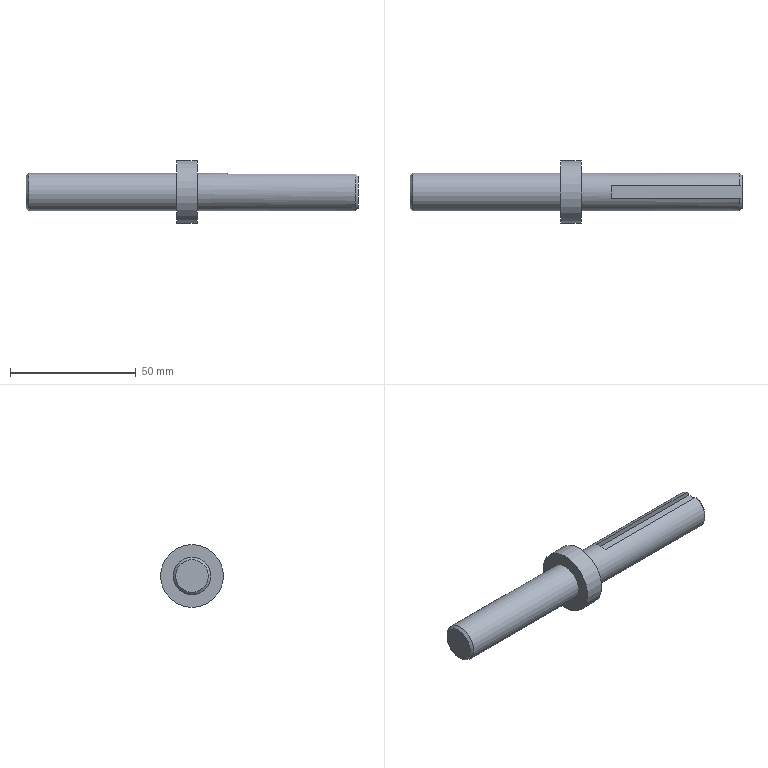Component | NX | SCREW_4_1 | 1 solid | 13 faces | box 132 x 25 x 25 mm | volume 25184 mm3 | plane 8 | cylinder 3 | cone 2 | commonest cylinder face diameters 15 x2 25 x1
STEP:
#1=CARTESIAN_POINT('',(0.,0.,0.));
#2=DIRECTION('',(0.,0.,1.));
#3=DIRECTION('',(1.,0.,0.));
#4=AXIS2_PLACEMENT_3D('',#1,#2,#3);
#5=CARTESIAN_POINT('',(209.,-2.5,107.5));
#6=VERTEX_POINT('',#5);
#7=CARTESIAN_POINT('',(209.,-2.5,108.5));
#8=VERTEX_POINT('',#7);
#9=CARTESIAN_POINT('',(209.,-2.5,102.5));
#10=DIRECTION('',(0.,0.,1.));
#11=VECTOR('',#10,1.);
#12=LINE('',#9,#11);
#13=CARTESIAN_POINT('',(209.,0.,102.5));
#14=DIRECTION('',(1.,0.,0.));
#15=DIRECTION('',(0.,0.,1.));
#16=AXIS2_PLACEMENT_3D('',#13,#14,#15);
#17=PLANE('',#16);
#18=CARTESIAN_POINT('',(0.,2.5));
#19=DIRECTION('',(1.,0.));
#20=VECTOR('',#19,1.);
#21=LINE('',#18,#20);
#22=(GEOMETRIC_REPRESENTATION_CONTEXT(2)PARAMETRIC_REPRESENTATION_CONTEXT()REPRESENTATION_CONTEXT('',''));
#23=DEFINITIONAL_REPRESENTATION('',(#21),#22);
#24=PCURVE('',#17,#23);
#25=CARTESIAN_POINT('',(77.,-2.5,102.5));
#26=DIRECTION('',(0.,1.,0.));
#27=DIRECTION('',(0.,0.,1.));
#28=AXIS2_PLACEMENT_3D('',#25,#26,#27);
#29=PLANE('',#28);
#30=CARTESIAN_POINT('',(0.,132.));
#31=DIRECTION('',(1.,0.));
#32=VECTOR('',#31,1.);
#33=LINE('',#30,#32);
#34=(GEOMETRIC_REPRESENTATION_CONTEXT(2)PARAMETRIC_REPRESENTATION_CONTEXT()REPRESENTATION_CONTEXT('',''));
#35=DEFINITIONAL_REPRESENTATION('',(#33),#34);
#36=PCURVE('',#29,#35);
#37=SURFACE_CURVE('',#12,(#24,#36),.PCURVE_S1.);
#38=EDGE_CURVE('',#6,#8,#37,.T.);
#39=ORIENTED_EDGE('',*,*,#38,.T.);
#40=CARTESIAN_POINT('',(209.,2.5,108.5));
#41=VERTEX_POINT('',#40);
#42=CARTESIAN_POINT('',(209.,0.,102.5));
#43=DIRECTION('',(1.,0.,0.));
#44=DIRECTION('',(0.,0.,1.));
#45=AXIS2_PLACEMENT_3D('',#42,#43,#44);
#46=CIRCLE('',#45,6.5);
#47=CARTESIAN_POINT('',(0.,0.));
#48=DIRECTION('',(1.,0.));
#49=AXIS2_PLACEMENT_2D('',#47,#48);
#50=CIRCLE('',#49,6.5);
#51=(GEOMETRIC_REPRESENTATION_CONTEXT(2)PARAMETRIC_REPRESENTATION_CONTEXT()REPRESENTATION_CONTEXT('',''));
#52=DEFINITIONAL_REPRESENTATION('',(#50),#51);
#53=PCURVE('',#17,#52);
#54=CARTESIAN_POINT('',(209.,0.,102.5));
#55=DIRECTION('',(-1.,0.,0.));
#56=DIRECTION('',(0.,0.,-1.));
#57=AXIS2_PLACEMENT_3D('',#54,#55,#56);
#58=CONICAL_SURFACE('',#57,6.5,0.7854);
#59=CARTESIAN_POINT('',(3.142,-0.));
#60=DIRECTION('',(-1.,0.));
#61=VECTOR('',#60,1.);
#62=LINE('',#59,#61);
#63=(GEOMETRIC_REPRESENTATION_CONTEXT(2)PARAMETRIC_REPRESENTATION_CONTEXT()REPRESENTATION_CONTEXT('',''));
#64=DEFINITIONAL_REPRESENTATION('',(#62),#63);
#65=PCURVE('',#58,#64);
#66=SURFACE_CURVE('',#46,(#53,#65),.PCURVE_S1.);
#67=EDGE_CURVE('',#8,#41,#66,.T.);
#68=ORIENTED_EDGE('',*,*,#67,.T.);
#69=CARTESIAN_POINT('',(209.,2.5,107.5));
#70=VERTEX_POINT('',#69);
#71=CARTESIAN_POINT('',(209.,2.5,102.5));
#72=DIRECTION('',(0.,0.,-1.));
#73=VECTOR('',#72,1.);
#74=LINE('',#71,#73);
#75=CARTESIAN_POINT('',(0.,-2.5));
#76=DIRECTION('',(-1.,0.));
#77=VECTOR('',#76,1.);
#78=LINE('',#75,#77);
#79=(GEOMETRIC_REPRESENTATION_CONTEXT(2)PARAMETRIC_REPRESENTATION_CONTEXT()REPRESENTATION_CONTEXT('',''));
#80=DEFINITIONAL_REPRESENTATION('',(#78),#79);
#81=PCURVE('',#17,#80);
#82=CARTESIAN_POINT('',(77.,2.5,102.5));
#83=DIRECTION('',(0.,1.,0.));
#84=DIRECTION('',(0.,0.,1.));
#85=AXIS2_PLACEMENT_3D('',#82,#83,#84);
#86=PLANE('',#85);
#87=CARTESIAN_POINT('',(0.,132.));
#88=DIRECTION('',(-1.,0.));
#89=VECTOR('',#88,1.);
#90=LINE('',#87,#89);
#91=(GEOMETRIC_REPRESENTATION_CONTEXT(2)PARAMETRIC_REPRESENTATION_CONTEXT()REPRESENTATION_CONTEXT('',''));
#92=DEFINITIONAL_REPRESENTATION('',(#90),#91);
#93=PCURVE('',#86,#92);
#94=SURFACE_CURVE('',#74,(#81,#93),.PCURVE_S1.);
#95=EDGE_CURVE('',#41,#70,#94,.T.);
#96=ORIENTED_EDGE('',*,*,#95,.T.);
#97=CARTESIAN_POINT('',(209.,0.,107.5));
#98=DIRECTION('',(0.,1.,0.));
#99=VECTOR('',#98,1.);
#100=LINE('',#97,#99);
#101=CARTESIAN_POINT('',(5.,0.));
#102=DIRECTION('',(0.,-1.));
#103=VECTOR('',#102,1.);
#104=LINE('',#101,#103);
#105=(GEOMETRIC_REPRESENTATION_CONTEXT(2)PARAMETRIC_REPRESENTATION_CONTEXT()REPRESENTATION_CONTEXT('',''));
#106=DEFINITIONAL_REPRESENTATION('',(#104),#105);
#107=PCURVE('',#17,#106);
#108=CARTESIAN_POINT('',(192.,-2.5,107.5));
#109=DIRECTION('',(-0.,0.,-1.));
#110=DIRECTION('',(1.,0.,-0.));
#111=AXIS2_PLACEMENT_3D('',#108,#109,#110);
#112=PLANE('',#111);
#113=CARTESIAN_POINT('',(17.,-2.5));
#114=DIRECTION('',(0.,-1.));
#115=VECTOR('',#114,1.);
#116=LINE('',#113,#115);
#117=(GEOMETRIC_REPRESENTATION_CONTEXT(2)PARAMETRIC_REPRESENTATION_CONTEXT()REPRESENTATION_CONTEXT('',''));
#118=DEFINITIONAL_REPRESENTATION('',(#116),#117);
#119=PCURVE('',#112,#118);
#120=SURFACE_CURVE('',#100,(#107,#119),.PCURVE_S1.);
#121=EDGE_CURVE('',#6,#70,#120,.T.);
#122=ORIENTED_EDGE('',*,*,#121,.F.);
#123=EDGE_LOOP('',(#39,#68,#96,#122));
#124=FACE_BOUND('',#123,.T.);
#125=ADVANCED_FACE('',(#124),#17,.T.);
#126=ORIENTED_EDGE('',*,*,#95,.F.);
#127=CARTESIAN_POINT('',(208.,2.5,109.571));
#128=VERTEX_POINT('',#127);
#129=CARTESIAN_POINT('',(209.,2.5,108.5));
#130=CARTESIAN_POINT('',(208.669,2.5,108.859));
#131=CARTESIAN_POINT('',(208.335,2.5,109.216));
#132=CARTESIAN_POINT('',(208.,2.5,109.571));
#133=B_SPLINE_CURVE_WITH_KNOTS('',3,(#129,#130,#131,#132),.UNSPECIFIED.,.F.,.F.,(4,4),(0.,1.),.PIECEWISE_BEZIER_KNOTS.);
#134=CARTESIAN_POINT('',(6.,132.));
#135=CARTESIAN_POINT('',(6.359,131.669));
#136=CARTESIAN_POINT('',(6.716,131.335));
#137=CARTESIAN_POINT('',(7.071,131.));
#138=B_SPLINE_CURVE_WITH_KNOTS('',3,(#134,#135,#136,#137),.UNSPECIFIED.,.F.,.F.,(4,4),(0.,1.),.PIECEWISE_BEZIER_KNOTS.);
#139=(GEOMETRIC_REPRESENTATION_CONTEXT(2)PARAMETRIC_REPRESENTATION_CONTEXT()REPRESENTATION_CONTEXT('',''));
#140=DEFINITIONAL_REPRESENTATION('',(#138),#139);
#141=PCURVE('',#86,#140);
#142=CARTESIAN_POINT('',(-2.747,0.));
#143=CARTESIAN_POINT('',(-2.802,1.));
#144=B_SPLINE_CURVE_WITH_KNOTS('',1,(#142,#143),.UNSPECIFIED.,.F.,.F.,(2,2),(0.,1.),.PIECEWISE_BEZIER_KNOTS.);
#145=(GEOMETRIC_REPRESENTATION_CONTEXT(2)PARAMETRIC_REPRESENTATION_CONTEXT()REPRESENTATION_CONTEXT('',''));
#146=DEFINITIONAL_REPRESENTATION('',(#144),#145);
#147=PCURVE('',#58,#146);
#148=SURFACE_CURVE('',#133,(#141,#147),.PCURVE_S1.);
#149=EDGE_CURVE('',#41,#128,#148,.T.);
#150=ORIENTED_EDGE('',*,*,#149,.T.);
#151=CARTESIAN_POINT('',(157.,2.5,109.571));
#152=VERTEX_POINT('',#151);
#153=CARTESIAN_POINT('',(74.99,2.5,109.571));
#154=DIRECTION('',(-1.,0.,0.));
#155=VECTOR('',#154,1.);
#156=LINE('',#153,#155);
#157=CARTESIAN_POINT('',(7.071,-2.01));
#158=DIRECTION('',(0.,-1.));
#159=VECTOR('',#158,1.);
#160=LINE('',#157,#159);
#161=(GEOMETRIC_REPRESENTATION_CONTEXT(2)PARAMETRIC_REPRESENTATION_CONTEXT()REPRESENTATION_CONTEXT('',''));
#162=DEFINITIONAL_REPRESENTATION('',(#160),#161);
#163=PCURVE('',#86,#162);
#164=CARTESIAN_POINT('',(74.99,0.,102.5));
#165=DIRECTION('',(1.,0.,0.));
#166=DIRECTION('',(0.,0.,1.));
#167=AXIS2_PLACEMENT_3D('',#164,#165,#166);
#168=CYLINDRICAL_SURFACE('',#167,7.5);
#169=CARTESIAN_POINT('',(5.943,0.));
#170=DIRECTION('',(0.,-1.));
#171=VECTOR('',#170,1.);
#172=LINE('',#169,#171);
#173=(GEOMETRIC_REPRESENTATION_CONTEXT(2)PARAMETRIC_REPRESENTATION_CONTEXT()REPRESENTATION_CONTEXT('',''));
#174=DEFINITIONAL_REPRESENTATION('',(#172),#173);
#175=PCURVE('',#168,#174);
#176=SURFACE_CURVE('',#156,(#163,#175),.PCURVE_S1.);
#177=EDGE_CURVE('',#128,#152,#176,.T.);
#178=ORIENTED_EDGE('',*,*,#177,.T.);
#179=CARTESIAN_POINT('',(157.,2.5,107.5));
#180=VERTEX_POINT('',#179);
#181=CARTESIAN_POINT('',(157.,2.5,107.5));
#182=DIRECTION('',(0.,0.,-1.));
#183=VECTOR('',#182,1.);
#184=LINE('',#181,#183);
#185=CARTESIAN_POINT('',(5.,80.));
#186=DIRECTION('',(-1.,0.));
#187=VECTOR('',#186,1.);
#188=LINE('',#185,#187);
#189=(GEOMETRIC_REPRESENTATION_CONTEXT(2)PARAMETRIC_REPRESENTATION_CONTEXT()REPRESENTATION_CONTEXT('',''));
#190=DEFINITIONAL_REPRESENTATION('',(#188),#189);
#191=PCURVE('',#86,#190);
#192=CARTESIAN_POINT('',(157.,-2.5,107.5));
#193=DIRECTION('',(-1.,0.,0.));
#194=DIRECTION('',(0.,0.,-1.));
#195=AXIS2_PLACEMENT_3D('',#192,#193,#194);
#196=PLANE('',#195);
#197=CARTESIAN_POINT('',(0.,-5.));
#198=DIRECTION('',(1.,0.));
#199=VECTOR('',#198,1.);
#200=LINE('',#197,#199);
#201=(GEOMETRIC_REPRESENTATION_CONTEXT(2)PARAMETRIC_REPRESENTATION_CONTEXT()REPRESENTATION_CONTEXT('',''));
#202=DEFINITIONAL_REPRESENTATION('',(#200),#201);
#203=PCURVE('',#196,#202);
#204=SURFACE_CURVE('',#184,(#191,#203),.PCURVE_S1.);
#205=EDGE_CURVE('',#152,#180,#204,.T.);
#206=ORIENTED_EDGE('',*,*,#205,.T.);
#207=CARTESIAN_POINT('',(192.,2.5,107.5));
#208=DIRECTION('',(1.,0.,-0.));
#209=VECTOR('',#208,1.);
#210=LINE('',#207,#209);
#211=CARTESIAN_POINT('',(5.,115.));
#212=DIRECTION('',(-0.,1.));
#213=VECTOR('',#212,1.);
#214=LINE('',#211,#213);
#215=(GEOMETRIC_REPRESENTATION_CONTEXT(2)PARAMETRIC_REPRESENTATION_CONTEXT()REPRESENTATION_CONTEXT('',''));
#216=DEFINITIONAL_REPRESENTATION('',(#214),#215);
#217=PCURVE('',#86,#216);
#218=CARTESIAN_POINT('',(0.,-5.));
#219=DIRECTION('',(1.,0.));
#220=VECTOR('',#219,1.);
#221=LINE('',#218,#220);
#222=(GEOMETRIC_REPRESENTATION_CONTEXT(2)PARAMETRIC_REPRESENTATION_CONTEXT()REPRESENTATION_CONTEXT('',''));
#223=DEFINITIONAL_REPRESENTATION('',(#221),#222);
#224=PCURVE('',#112,#223);
#225=SURFACE_CURVE('',#210,(#217,#224),.PCURVE_S1.);
#226=EDGE_CURVE('',#180,#70,#225,.T.);
#227=ORIENTED_EDGE('',*,*,#226,.T.);
#228=EDGE_LOOP('',(#126,#150,#178,#206,#227));
#229=FACE_BOUND('',#228,.T.);
#230=ADVANCED_FACE('',(#229),#86,.F.);
#231=CARTESIAN_POINT('',(77.,0.,96.));
#232=VERTEX_POINT('',#231);
#233=CARTESIAN_POINT('',(77.,0.,102.5));
#234=DIRECTION('',(-1.,0.,0.));
#235=DIRECTION('',(0.,0.,-1.));
#236=AXIS2_PLACEMENT_3D('',#233,#234,#235);
#237=CIRCLE('',#236,6.5);
#238=CARTESIAN_POINT('',(77.,0.,110.));
#239=DIRECTION('',(-1.,0.,0.));
#240=DIRECTION('',(0.,0.,-1.));
#241=AXIS2_PLACEMENT_3D('',#238,#239,#240);
#242=PLANE('',#241);
#243=CARTESIAN_POINT('',(7.5,0.));
#244=DIRECTION('',(1.,0.));
#245=AXIS2_PLACEMENT_2D('',#243,#244);
#246=CIRCLE('',#245,6.5);
#247=(GEOMETRIC_REPRESENTATION_CONTEXT(2)PARAMETRIC_REPRESENTATION_CONTEXT()REPRESENTATION_CONTEXT('',''));
#248=DEFINITIONAL_REPRESENTATION('',(#246),#247);
#249=PCURVE('',#242,#248);
#250=CARTESIAN_POINT('',(78.,0.,102.5));
#251=DIRECTION('',(1.,0.,0.));
#252=DIRECTION('',(0.,0.,1.));
#253=AXIS2_PLACEMENT_3D('',#250,#251,#252);
#254=CONICAL_SURFACE('',#253,7.5,0.7854);
#255=CARTESIAN_POINT('',(9.425,-1.));
#256=DIRECTION('',(-1.,0.));
#257=VECTOR('',#256,1.);
#258=LINE('',#255,#257);
#259=(GEOMETRIC_REPRESENTATION_CONTEXT(2)PARAMETRIC_REPRESENTATION_CONTEXT()REPRESENTATION_CONTEXT('',''));
#260=DEFINITIONAL_REPRESENTATION('',(#258),#259);
#261=PCURVE('',#254,#260);
#262=SURFACE_CURVE('',#237,(#249,#261),.PCURVE_S1.);
#263=EDGE_CURVE('',#232,#232,#262,.T.);
#264=ORIENTED_EDGE('',*,*,#263,.T.);
#265=EDGE_LOOP('',(#264));
#266=FACE_BOUND('',#265,.T.);
#267=ADVANCED_FACE('',(#266),#242,.T.);
#268=CARTESIAN_POINT('',(78.,0.,95.));
#269=VERTEX_POINT('',#268);
#270=CARTESIAN_POINT('',(78.,0.,110.));
#271=VERTEX_POINT('',#270);
#272=CARTESIAN_POINT('',(78.,0.,102.5));
#273=DIRECTION('',(1.,0.,0.));
#274=DIRECTION('',(0.,0.,-1.));
#275=AXIS2_PLACEMENT_3D('',#272,#273,#274);
#276=CIRCLE('',#275,7.5);
#277=CARTESIAN_POINT('',(74.99,0.,102.5));
#278=DIRECTION('',(1.,0.,0.));
#279=DIRECTION('',(0.,0.,1.));
#280=AXIS2_PLACEMENT_3D('',#277,#278,#279);
#281=CYLINDRICAL_SURFACE('',#280,7.5);
#282=CARTESIAN_POINT('',(3.142,3.01));
#283=DIRECTION('',(1.,0.));
#284=VECTOR('',#283,1.);
#285=LINE('',#282,#284);
#286=(GEOMETRIC_REPRESENTATION_CONTEXT(2)PARAMETRIC_REPRESENTATION_CONTEXT()REPRESENTATION_CONTEXT('',''));
#287=DEFINITIONAL_REPRESENTATION('',(#285),#286);
#288=PCURVE('',#281,#287);
#289=CARTESIAN_POINT('',(3.142,0.));
#290=DIRECTION('',(1.,0.));
#291=VECTOR('',#290,1.);
#292=LINE('',#289,#291);
#293=(GEOMETRIC_REPRESENTATION_CONTEXT(2)PARAMETRIC_REPRESENTATION_CONTEXT()REPRESENTATION_CONTEXT('',''));
#294=DEFINITIONAL_REPRESENTATION('',(#292),#293);
#295=PCURVE('',#254,#294);
#296=SURFACE_CURVE('',#276,(#288,#295),.PCURVE_S1.);
#297=EDGE_CURVE('',#269,#271,#296,.T.);
#298=ORIENTED_EDGE('',*,*,#297,.T.);
#299=CARTESIAN_POINT('',(137.,0.,110.));
#300=VERTEX_POINT('',#299);
#301=CARTESIAN_POINT('',(78.,0.,110.));
#302=CARTESIAN_POINT('',(137.,0.,110.));
#303=B_SPLINE_CURVE_WITH_KNOTS('',1,(#301,#302),.UNSPECIFIED.,.F.,.F.,(2,2),(3.01,62.01),.PIECEWISE_BEZIER_KNOTS.);
#304=CARTESIAN_POINT('',(6.283,0.));
#305=DIRECTION('',(0.,1.));
#306=VECTOR('',#305,1.);
#307=LINE('',#304,#306);
#308=(GEOMETRIC_REPRESENTATION_CONTEXT(2)PARAMETRIC_REPRESENTATION_CONTEXT()REPRESENTATION_CONTEXT('',''));
#309=DEFINITIONAL_REPRESENTATION('',(#307),#308);
#310=PCURVE('',#281,#309);
#311=CARTESIAN_POINT('',(0.,0.));
#312=DIRECTION('',(0.,1.));
#313=VECTOR('',#312,1.);
#314=LINE('',#311,#313);
#315=(GEOMETRIC_REPRESENTATION_CONTEXT(2)PARAMETRIC_REPRESENTATION_CONTEXT()REPRESENTATION_CONTEXT('',''));
#316=DEFINITIONAL_REPRESENTATION('',(#314),#315);
#317=PCURVE('',#281,#316);
#318=SEAM_CURVE('',#303,(#310,#317),.PCURVE_S1.);
#319=EDGE_CURVE('',#271,#300,#318,.T.);
#320=ORIENTED_EDGE('',*,*,#319,.T.);
#321=CARTESIAN_POINT('',(137.,0.,102.5));
#322=DIRECTION('',(1.,0.,0.));
#323=DIRECTION('',(0.,0.,1.));
#324=AXIS2_PLACEMENT_3D('',#321,#322,#323);
#325=CIRCLE('',#324,7.5);
#326=CARTESIAN_POINT('',(0.,62.01));
#327=DIRECTION('',(1.,0.));
#328=VECTOR('',#327,1.);
#329=LINE('',#326,#328);
#330=(GEOMETRIC_REPRESENTATION_CONTEXT(2)PARAMETRIC_REPRESENTATION_CONTEXT()REPRESENTATION_CONTEXT('',''));
#331=DEFINITIONAL_REPRESENTATION('',(#329),#330);
#332=PCURVE('',#281,#331);
#333=CARTESIAN_POINT('',(137.,0.,115.));
#334=DIRECTION('',(-1.,0.,0.));
#335=DIRECTION('',(0.,0.,-1.));
#336=AXIS2_PLACEMENT_3D('',#333,#334,#335);
#337=PLANE('',#336);
#338=CARTESIAN_POINT('',(5.,0.));
#339=CARTESIAN_POINT('',(5.,12.99));
#340=CARTESIAN_POINT('',(16.25,6.495));
#341=CARTESIAN_POINT('',(27.5,0.));
#342=CARTESIAN_POINT('',(16.25,-6.495));
#343=CARTESIAN_POINT('',(5.,-12.99));
#344=CARTESIAN_POINT('',(5.,0.));
#345=(BOUNDED_CURVE()B_SPLINE_CURVE(2,(#338,#339,#340,#341,#342,#343,#344),.UNSPECIFIED.,.T.,.F.)B_SPLINE_CURVE_WITH_KNOTS((1,2,2,2,2,1),(-2.094,0.,2.094,4.189,6.283,8.378),.UNSPECIFIED.)CURVE()GEOMETRIC_REPRESENTATION_ITEM()RATIONAL_B_SPLINE_CURVE((1.,0.5,1.,0.5,1.,0.5,1.))REPRESENTATION_ITEM(''));
#346=(GEOMETRIC_REPRESENTATION_CONTEXT(2)PARAMETRIC_REPRESENTATION_CONTEXT()REPRESENTATION_CONTEXT('',''));
#347=DEFINITIONAL_REPRESENTATION('',(#345),#346);
#348=PCURVE('',#337,#347);
#349=SURFACE_CURVE('',#325,(#332,#348),.PCURVE_S1.);
#350=EDGE_CURVE('',#300,#300,#349,.T.);
#351=ORIENTED_EDGE('',*,*,#350,.F.);
#352=ORIENTED_EDGE('',*,*,#319,.F.);
#353=CARTESIAN_POINT('',(78.,0.,102.5));
#354=DIRECTION('',(1.,0.,0.));
#355=DIRECTION('',(0.,0.,-1.));
#356=AXIS2_PLACEMENT_3D('',#353,#354,#355);
#357=CIRCLE('',#356,7.5);
#358=CARTESIAN_POINT('',(-3.142,3.01));
#359=DIRECTION('',(1.,0.));
#360=VECTOR('',#359,1.);
#361=LINE('',#358,#360);
#362=(GEOMETRIC_REPRESENTATION_CONTEXT(2)PARAMETRIC_REPRESENTATION_CONTEXT()REPRESENTATION_CONTEXT('',''));
#363=DEFINITIONAL_REPRESENTATION('',(#361),#362);
#364=PCURVE('',#281,#363);
#365=CARTESIAN_POINT('',(3.142,0.));
#366=DIRECTION('',(1.,0.));
#367=VECTOR('',#366,1.);
#368=LINE('',#365,#367);
#369=(GEOMETRIC_REPRESENTATION_CONTEXT(2)PARAMETRIC_REPRESENTATION_CONTEXT()REPRESENTATION_CONTEXT('',''));
#370=DEFINITIONAL_REPRESENTATION('',(#368),#369);
#371=PCURVE('',#254,#370);
#372=SURFACE_CURVE('',#357,(#364,#371),.PCURVE_S1.);
#373=EDGE_CURVE('',#271,#269,#372,.T.);
#374=ORIENTED_EDGE('',*,*,#373,.T.);
#375=EDGE_LOOP('',(#298,#320,#351,#352,#374));
#376=FACE_BOUND('',#375,.T.);
#377=ADVANCED_FACE('',(#376),#281,.T.);
#378=ORIENTED_EDGE('',*,*,#350,.T.);
#379=EDGE_LOOP('',(#378));
#380=FACE_BOUND('',#379,.T.);
#381=CARTESIAN_POINT('',(137.,0.,115.));
#382=VERTEX_POINT('',#381);
#383=CARTESIAN_POINT('',(137.,0.,102.5));
#384=DIRECTION('',(1.,0.,0.));
#385=DIRECTION('',(0.,0.,1.));
#386=AXIS2_PLACEMENT_3D('',#383,#384,#385);
#387=CIRCLE('',#386,12.5);
#388=CARTESIAN_POINT('',(0.,0.));
#389=CARTESIAN_POINT('',(0.,21.651));
#390=CARTESIAN_POINT('',(18.75,10.825));
#391=CARTESIAN_POINT('',(37.5,0.));
#392=CARTESIAN_POINT('',(18.75,-10.825));
#393=CARTESIAN_POINT('',(0.,-21.651));
#394=CARTESIAN_POINT('',(0.,0.));
#395=(BOUNDED_CURVE()B_SPLINE_CURVE(2,(#388,#389,#390,#391,#392,#393,#394),.UNSPECIFIED.,.T.,.F.)B_SPLINE_CURVE_WITH_KNOTS((1,2,2,2,2,1),(-2.094,0.,2.094,4.189,6.283,8.378),.UNSPECIFIED.)CURVE()GEOMETRIC_REPRESENTATION_ITEM()RATIONAL_B_SPLINE_CURVE((1.,0.5,1.,0.5,1.,0.5,1.))REPRESENTATION_ITEM(''));
#396=(GEOMETRIC_REPRESENTATION_CONTEXT(2)PARAMETRIC_REPRESENTATION_CONTEXT()REPRESENTATION_CONTEXT('',''));
#397=DEFINITIONAL_REPRESENTATION('',(#395),#396);
#398=PCURVE('',#337,#397);
#399=CARTESIAN_POINT('',(74.99,0.,102.5));
#400=DIRECTION('',(1.,0.,0.));
#401=DIRECTION('',(0.,0.,1.));
#402=AXIS2_PLACEMENT_3D('',#399,#400,#401);
#403=CYLINDRICAL_SURFACE('',#402,12.5);
#404=CARTESIAN_POINT('',(0.,62.01));
#405=DIRECTION('',(1.,0.));
#406=VECTOR('',#405,1.);
#407=LINE('',#404,#406);
#408=(GEOMETRIC_REPRESENTATION_CONTEXT(2)PARAMETRIC_REPRESENTATION_CONTEXT()REPRESENTATION_CONTEXT('',''));
#409=DEFINITIONAL_REPRESENTATION('',(#407),#408);
#410=PCURVE('',#403,#409);
#411=SURFACE_CURVE('',#387,(#398,#410),.PCURVE_S1.);
#412=EDGE_CURVE('',#382,#382,#411,.T.);
#413=ORIENTED_EDGE('',*,*,#412,.F.);
#414=EDGE_LOOP('',(#413));
#415=FACE_BOUND('',#414,.T.);
#416=ADVANCED_FACE('',(#380,#415),#337,.T.);
#417=ORIENTED_EDGE('',*,*,#412,.T.);
#418=CARTESIAN_POINT('',(145.,0.,115.));
#419=VERTEX_POINT('',#418);
#420=CARTESIAN_POINT('',(137.,0.,115.));
#421=CARTESIAN_POINT('',(145.,0.,115.));
#422=B_SPLINE_CURVE_WITH_KNOTS('',1,(#420,#421),.UNSPECIFIED.,.F.,.F.,(2,2),(62.01,70.01),.PIECEWISE_BEZIER_KNOTS.);
#423=CARTESIAN_POINT('',(6.283,0.));
#424=DIRECTION('',(0.,1.));
#425=VECTOR('',#424,1.);
#426=LINE('',#423,#425);
#427=(GEOMETRIC_REPRESENTATION_CONTEXT(2)PARAMETRIC_REPRESENTATION_CONTEXT()REPRESENTATION_CONTEXT('',''));
#428=DEFINITIONAL_REPRESENTATION('',(#426),#427);
#429=PCURVE('',#403,#428);
#430=CARTESIAN_POINT('',(0.,0.));
#431=DIRECTION('',(0.,1.));
#432=VECTOR('',#431,1.);
#433=LINE('',#430,#432);
#434=(GEOMETRIC_REPRESENTATION_CONTEXT(2)PARAMETRIC_REPRESENTATION_CONTEXT()REPRESENTATION_CONTEXT('',''));
#435=DEFINITIONAL_REPRESENTATION('',(#433),#434);
#436=PCURVE('',#403,#435);
#437=SEAM_CURVE('',#422,(#429,#436),.PCURVE_S1.);
#438=EDGE_CURVE('',#382,#419,#437,.T.);
#439=ORIENTED_EDGE('',*,*,#438,.T.);
#440=CARTESIAN_POINT('',(145.,0.,102.5));
#441=DIRECTION('',(1.,0.,0.));
#442=DIRECTION('',(0.,0.,1.));
#443=AXIS2_PLACEMENT_3D('',#440,#441,#442);
#444=CIRCLE('',#443,12.5);
#445=CARTESIAN_POINT('',(0.,70.01));
#446=DIRECTION('',(1.,0.));
#447=VECTOR('',#446,1.);
#448=LINE('',#445,#447);
#449=(GEOMETRIC_REPRESENTATION_CONTEXT(2)PARAMETRIC_REPRESENTATION_CONTEXT()REPRESENTATION_CONTEXT('',''));
#450=DEFINITIONAL_REPRESENTATION('',(#448),#449);
#451=PCURVE('',#403,#450);
#452=CARTESIAN_POINT('',(145.,0.,110.));
#453=DIRECTION('',(1.,0.,0.));
#454=DIRECTION('',(0.,0.,1.));
#455=AXIS2_PLACEMENT_3D('',#452,#453,#454);
#456=PLANE('',#455);
#457=CARTESIAN_POINT('',(-7.5,0.));
#458=DIRECTION('',(1.,0.));
#459=AXIS2_PLACEMENT_2D('',#457,#458);
#460=CIRCLE('',#459,12.5);
#461=(GEOMETRIC_REPRESENTATION_CONTEXT(2)PARAMETRIC_REPRESENTATION_CONTEXT()REPRESENTATION_CONTEXT('',''));
#462=DEFINITIONAL_REPRESENTATION('',(#460),#461);
#463=PCURVE('',#456,#462);
#464=SURFACE_CURVE('',#444,(#451,#463),.PCURVE_S1.);
#465=EDGE_CURVE('',#419,#419,#464,.T.);
#466=ORIENTED_EDGE('',*,*,#465,.F.);
#467=ORIENTED_EDGE('',*,*,#438,.F.);
#468=EDGE_LOOP('',(#417,#439,#466,#467));
#469=FACE_BOUND('',#468,.T.);
#470=ADVANCED_FACE('',(#469),#403,.T.);
#471=ORIENTED_EDGE('',*,*,#465,.T.);
#472=EDGE_LOOP('',(#471));
#473=FACE_BOUND('',#472,.T.);
#474=CARTESIAN_POINT('',(145.,0.,110.));
#475=VERTEX_POINT('',#474);
#476=CARTESIAN_POINT('',(145.,0.,102.5));
#477=DIRECTION('',(1.,0.,0.));
#478=DIRECTION('',(0.,0.,1.));
#479=AXIS2_PLACEMENT_3D('',#476,#477,#478);
#480=CIRCLE('',#479,7.5);
#481=CARTESIAN_POINT('',(-7.5,0.));
#482=DIRECTION('',(1.,0.));
#483=AXIS2_PLACEMENT_2D('',#481,#482);
#484=CIRCLE('',#483,7.5);
#485=(GEOMETRIC_REPRESENTATION_CONTEXT(2)PARAMETRIC_REPRESENTATION_CONTEXT()REPRESENTATION_CONTEXT('',''));
#486=DEFINITIONAL_REPRESENTATION('',(#484),#485);
#487=PCURVE('',#456,#486);
#488=CARTESIAN_POINT('',(0.,70.01));
#489=DIRECTION('',(1.,0.));
#490=VECTOR('',#489,1.);
#491=LINE('',#488,#490);
#492=(GEOMETRIC_REPRESENTATION_CONTEXT(2)PARAMETRIC_REPRESENTATION_CONTEXT()REPRESENTATION_CONTEXT('',''));
#493=DEFINITIONAL_REPRESENTATION('',(#491),#492);
#494=PCURVE('',#168,#493);
#495=SURFACE_CURVE('',#480,(#487,#494),.PCURVE_S1.);
#496=EDGE_CURVE('',#475,#475,#495,.T.);
#497=ORIENTED_EDGE('',*,*,#496,.F.);
#498=EDGE_LOOP('',(#497));
#499=FACE_BOUND('',#498,.T.);
#500=ADVANCED_FACE('',(#473,#499),#456,.T.);
#501=ORIENTED_EDGE('',*,*,#177,.F.);
#502=CARTESIAN_POINT('',(208.,-2.5,109.571));
#503=VERTEX_POINT('',#502);
#504=CARTESIAN_POINT('',(208.,0.,102.5));
#505=DIRECTION('',(-1.,0.,0.));
#506=DIRECTION('',(0.,0.,1.));
#507=AXIS2_PLACEMENT_3D('',#504,#505,#506);
#508=CIRCLE('',#507,7.5);
#509=CARTESIAN_POINT('',(6.283,133.01));
#510=DIRECTION('',(-1.,0.));
#511=VECTOR('',#510,1.);
#512=LINE('',#509,#511);
#513=(GEOMETRIC_REPRESENTATION_CONTEXT(2)PARAMETRIC_REPRESENTATION_CONTEXT()REPRESENTATION_CONTEXT('',''));
#514=DEFINITIONAL_REPRESENTATION('',(#512),#513);
#515=PCURVE('',#168,#514);
#516=CARTESIAN_POINT('',(-3.142,1.));
#517=DIRECTION('',(1.,0.));
#518=VECTOR('',#517,1.);
#519=LINE('',#516,#518);
#520=(GEOMETRIC_REPRESENTATION_CONTEXT(2)PARAMETRIC_REPRESENTATION_CONTEXT()REPRESENTATION_CONTEXT('',''));
#521=DEFINITIONAL_REPRESENTATION('',(#519),#520);
#522=PCURVE('',#58,#521);
#523=SURFACE_CURVE('',#508,(#515,#522),.PCURVE_S1.);
#524=EDGE_CURVE('',#128,#503,#523,.T.);
#525=ORIENTED_EDGE('',*,*,#524,.T.);
#526=CARTESIAN_POINT('',(157.,-2.5,109.571));
#527=VERTEX_POINT('',#526);
#528=CARTESIAN_POINT('',(74.99,-2.5,109.571));
#529=DIRECTION('',(-1.,0.,0.));
#530=VECTOR('',#529,1.);
#531=LINE('',#528,#530);
#532=CARTESIAN_POINT('',(0.3398,0.));
#533=DIRECTION('',(0.,-1.));
#534=VECTOR('',#533,1.);
#535=LINE('',#532,#534);
#536=(GEOMETRIC_REPRESENTATION_CONTEXT(2)PARAMETRIC_REPRESENTATION_CONTEXT()REPRESENTATION_CONTEXT('',''));
#537=DEFINITIONAL_REPRESENTATION('',(#535),#536);
#538=PCURVE('',#168,#537);
#539=CARTESIAN_POINT('',(7.071,-2.01));
#540=DIRECTION('',(0.,-1.));
#541=VECTOR('',#540,1.);
#542=LINE('',#539,#541);
#543=(GEOMETRIC_REPRESENTATION_CONTEXT(2)PARAMETRIC_REPRESENTATION_CONTEXT()REPRESENTATION_CONTEXT('',''));
#544=DEFINITIONAL_REPRESENTATION('',(#542),#543);
#545=PCURVE('',#29,#544);
#546=SURFACE_CURVE('',#531,(#538,#545),.PCURVE_S1.);
#547=EDGE_CURVE('',#503,#527,#546,.T.);
#548=ORIENTED_EDGE('',*,*,#547,.T.);
#549=CARTESIAN_POINT('',(157.,0.,110.));
#550=VERTEX_POINT('',#549);
#551=CARTESIAN_POINT('',(157.,0.,102.5));
#552=DIRECTION('',(1.,0.,0.));
#553=DIRECTION('',(0.,0.,-1.));
#554=AXIS2_PLACEMENT_3D('',#551,#552,#553);
#555=CIRCLE('',#554,7.5);
#556=CARTESIAN_POINT('',(-3.142,82.01));
#557=DIRECTION('',(1.,0.));
#558=VECTOR('',#557,1.);
#559=LINE('',#556,#558);
#560=(GEOMETRIC_REPRESENTATION_CONTEXT(2)PARAMETRIC_REPRESENTATION_CONTEXT()REPRESENTATION_CONTEXT('',''));
#561=DEFINITIONAL_REPRESENTATION('',(#559),#560);
#562=PCURVE('',#168,#561);
#563=CARTESIAN_POINT('',(12.5,-2.5));
#564=CARTESIAN_POINT('',(12.5,-15.49));
#565=CARTESIAN_POINT('',(1.25,-8.995));
#566=CARTESIAN_POINT('',(-10.,-2.5));
#567=CARTESIAN_POINT('',(1.25,3.995));
#568=CARTESIAN_POINT('',(12.5,10.49));
#569=CARTESIAN_POINT('',(12.5,-2.5));
#570=(BOUNDED_CURVE()B_SPLINE_CURVE(2,(#563,#564,#565,#566,#567,#568,#569),.UNSPECIFIED.,.T.,.F.)B_SPLINE_CURVE_WITH_KNOTS((1,2,2,2,2,1),(-2.094,0.,2.094,4.189,6.283,8.378),.UNSPECIFIED.)CURVE()GEOMETRIC_REPRESENTATION_ITEM()RATIONAL_B_SPLINE_CURVE((1.,0.5,1.,0.5,1.,0.5,1.))REPRESENTATION_ITEM(''));
#571=(GEOMETRIC_REPRESENTATION_CONTEXT(2)PARAMETRIC_REPRESENTATION_CONTEXT()REPRESENTATION_CONTEXT('',''));
#572=DEFINITIONAL_REPRESENTATION('',(#570),#571);
#573=PCURVE('',#196,#572);
#574=SURFACE_CURVE('',#555,(#562,#573),.PCURVE_S1.);
#575=EDGE_CURVE('',#550,#527,#574,.T.);
#576=ORIENTED_EDGE('',*,*,#575,.F.);
#577=CARTESIAN_POINT('',(145.,0.,110.));
#578=CARTESIAN_POINT('',(157.,0.,110.));
#579=B_SPLINE_CURVE_WITH_KNOTS('',1,(#577,#578),.UNSPECIFIED.,.F.,.F.,(2,2),(70.01,82.01),.PIECEWISE_BEZIER_KNOTS.);
#580=CARTESIAN_POINT('',(0.,0.));
#581=DIRECTION('',(0.,1.));
#582=VECTOR('',#581,1.);
#583=LINE('',#580,#582);
#584=(GEOMETRIC_REPRESENTATION_CONTEXT(2)PARAMETRIC_REPRESENTATION_CONTEXT()REPRESENTATION_CONTEXT('',''));
#585=DEFINITIONAL_REPRESENTATION('',(#583),#584);
#586=PCURVE('',#168,#585);
#587=CARTESIAN_POINT('',(6.283,0.));
#588=DIRECTION('',(0.,1.));
#589=VECTOR('',#588,1.);
#590=LINE('',#587,#589);
#591=(GEOMETRIC_REPRESENTATION_CONTEXT(2)PARAMETRIC_REPRESENTATION_CONTEXT()REPRESENTATION_CONTEXT('',''));
#592=DEFINITIONAL_REPRESENTATION('',(#590),#591);
#593=PCURVE('',#168,#592);
#594=SEAM_CURVE('',#579,(#586,#593),.PCURVE_S1.);
#595=EDGE_CURVE('',#475,#550,#594,.T.);
#596=ORIENTED_EDGE('',*,*,#595,.F.);
#597=ORIENTED_EDGE('',*,*,#496,.T.);
#598=ORIENTED_EDGE('',*,*,#595,.T.);
#599=CARTESIAN_POINT('',(157.,0.,102.5));
#600=DIRECTION('',(1.,0.,0.));
#601=DIRECTION('',(0.,0.,-1.));
#602=AXIS2_PLACEMENT_3D('',#599,#600,#601);
#603=CIRCLE('',#602,7.5);
#604=CARTESIAN_POINT('',(3.142,82.01));
#605=DIRECTION('',(1.,0.));
#606=VECTOR('',#605,1.);
#607=LINE('',#604,#606);
#608=(GEOMETRIC_REPRESENTATION_CONTEXT(2)PARAMETRIC_REPRESENTATION_CONTEXT()REPRESENTATION_CONTEXT('',''));
#609=DEFINITIONAL_REPRESENTATION('',(#607),#608);
#610=PCURVE('',#168,#609);
#611=CARTESIAN_POINT('',(12.5,-2.5));
#612=CARTESIAN_POINT('',(12.5,-15.49));
#613=CARTESIAN_POINT('',(1.25,-8.995));
#614=CARTESIAN_POINT('',(-10.,-2.5));
#615=CARTESIAN_POINT('',(1.25,3.995));
#616=CARTESIAN_POINT('',(12.5,10.49));
#617=CARTESIAN_POINT('',(12.5,-2.5));
#618=(BOUNDED_CURVE()B_SPLINE_CURVE(2,(#611,#612,#613,#614,#615,#616,#617),.UNSPECIFIED.,.T.,.F.)B_SPLINE_CURVE_WITH_KNOTS((1,2,2,2,2,1),(-2.094,0.,2.094,4.189,6.283,8.378),.UNSPECIFIED.)CURVE()GEOMETRIC_REPRESENTATION_ITEM()RATIONAL_B_SPLINE_CURVE((1.,0.5,1.,0.5,1.,0.5,1.))REPRESENTATION_ITEM(''));
#619=(GEOMETRIC_REPRESENTATION_CONTEXT(2)PARAMETRIC_REPRESENTATION_CONTEXT()REPRESENTATION_CONTEXT('',''));
#620=DEFINITIONAL_REPRESENTATION('',(#618),#619);
#621=PCURVE('',#196,#620);
#622=SURFACE_CURVE('',#603,(#610,#621),.PCURVE_S1.);
#623=EDGE_CURVE('',#152,#550,#622,.T.);
#624=ORIENTED_EDGE('',*,*,#623,.F.);
#625=EDGE_LOOP('',(#501,#525,#548,#576,#596,#597,#598,#624));
#626=FACE_BOUND('',#625,.T.);
#627=ADVANCED_FACE('',(#626),#168,.T.);
#628=ORIENTED_EDGE('',*,*,#205,.F.);
#629=ORIENTED_EDGE('',*,*,#623,.T.);
#630=ORIENTED_EDGE('',*,*,#575,.T.);
#631=CARTESIAN_POINT('',(157.,-2.5,107.5));
#632=VERTEX_POINT('',#631);
#633=CARTESIAN_POINT('',(157.,-2.5,107.5));
#634=DIRECTION('',(0.,0.,-1.));
#635=VECTOR('',#634,1.);
#636=LINE('',#633,#635);
#637=CARTESIAN_POINT('',(0.,0.));
#638=DIRECTION('',(1.,0.));
#639=VECTOR('',#638,1.);
#640=LINE('',#637,#639);
#641=(GEOMETRIC_REPRESENTATION_CONTEXT(2)PARAMETRIC_REPRESENTATION_CONTEXT()REPRESENTATION_CONTEXT('',''));
#642=DEFINITIONAL_REPRESENTATION('',(#640),#641);
#643=PCURVE('',#196,#642);
#644=CARTESIAN_POINT('',(5.,80.));
#645=DIRECTION('',(-1.,0.));
#646=VECTOR('',#645,1.);
#647=LINE('',#644,#646);
#648=(GEOMETRIC_REPRESENTATION_CONTEXT(2)PARAMETRIC_REPRESENTATION_CONTEXT()REPRESENTATION_CONTEXT('',''));
#649=DEFINITIONAL_REPRESENTATION('',(#647),#648);
#650=PCURVE('',#29,#649);
#651=SURFACE_CURVE('',#636,(#643,#650),.PCURVE_S1.);
#652=EDGE_CURVE('',#527,#632,#651,.T.);
#653=ORIENTED_EDGE('',*,*,#652,.T.);
#654=CARTESIAN_POINT('',(157.,-2.5,107.5));
#655=DIRECTION('',(0.,-1.,0.));
#656=VECTOR('',#655,1.);
#657=LINE('',#654,#656);
#658=CARTESIAN_POINT('',(0.,0.));
#659=DIRECTION('',(0.,1.));
#660=VECTOR('',#659,1.);
#661=LINE('',#658,#660);
#662=(GEOMETRIC_REPRESENTATION_CONTEXT(2)PARAMETRIC_REPRESENTATION_CONTEXT()REPRESENTATION_CONTEXT('',''));
#663=DEFINITIONAL_REPRESENTATION('',(#661),#662);
#664=PCURVE('',#196,#663);
#665=CARTESIAN_POINT('',(-35.,0.));
#666=DIRECTION('',(0.,1.));
#667=VECTOR('',#666,1.);
#668=LINE('',#665,#667);
#669=(GEOMETRIC_REPRESENTATION_CONTEXT(2)PARAMETRIC_REPRESENTATION_CONTEXT()REPRESENTATION_CONTEXT('',''));
#670=DEFINITIONAL_REPRESENTATION('',(#668),#669);
#671=PCURVE('',#112,#670);
#672=SURFACE_CURVE('',#657,(#664,#671),.PCURVE_S1.);
#673=EDGE_CURVE('',#180,#632,#672,.T.);
#674=ORIENTED_EDGE('',*,*,#673,.F.);
#675=EDGE_LOOP('',(#628,#629,#630,#653,#674));
#676=FACE_BOUND('',#675,.T.);
#677=ADVANCED_FACE('',(#676),#196,.F.);
#678=CARTESIAN_POINT('',(192.,-2.5,107.5));
#679=DIRECTION('',(1.,0.,-0.));
#680=VECTOR('',#679,1.);
#681=LINE('',#678,#680);
#682=CARTESIAN_POINT('',(0.,0.));
#683=DIRECTION('',(1.,0.));
#684=VECTOR('',#683,1.);
#685=LINE('',#682,#684);
#686=(GEOMETRIC_REPRESENTATION_CONTEXT(2)PARAMETRIC_REPRESENTATION_CONTEXT()REPRESENTATION_CONTEXT('',''));
#687=DEFINITIONAL_REPRESENTATION('',(#685),#686);
#688=PCURVE('',#112,#687);
#689=CARTESIAN_POINT('',(5.,115.));
#690=DIRECTION('',(-0.,1.));
#691=VECTOR('',#690,1.);
#692=LINE('',#689,#691);
#693=(GEOMETRIC_REPRESENTATION_CONTEXT(2)PARAMETRIC_REPRESENTATION_CONTEXT()REPRESENTATION_CONTEXT('',''));
#694=DEFINITIONAL_REPRESENTATION('',(#692),#693);
#695=PCURVE('',#29,#694);
#696=SURFACE_CURVE('',#681,(#688,#695),.PCURVE_S1.);
#697=EDGE_CURVE('',#632,#6,#696,.T.);
#698=ORIENTED_EDGE('',*,*,#697,.T.);
#699=ORIENTED_EDGE('',*,*,#121,.T.);
#700=ORIENTED_EDGE('',*,*,#226,.F.);
#701=ORIENTED_EDGE('',*,*,#673,.T.);
#702=EDGE_LOOP('',(#698,#699,#700,#701));
#703=FACE_BOUND('',#702,.T.);
#704=ADVANCED_FACE('',(#703),#112,.F.);
#705=ORIENTED_EDGE('',*,*,#547,.F.);
#706=CARTESIAN_POINT('',(208.,-2.5,109.571));
#707=CARTESIAN_POINT('',(208.335,-2.5,109.216));
#708=CARTESIAN_POINT('',(208.669,-2.5,108.859));
#709=CARTESIAN_POINT('',(209.,-2.5,108.5));
#710=B_SPLINE_CURVE_WITH_KNOTS('',3,(#706,#707,#708,#709),.UNSPECIFIED.,.F.,.F.,(4,4),(0.,1.),.PIECEWISE_BEZIER_KNOTS.);
#711=CARTESIAN_POINT('',(7.071,131.));
#712=CARTESIAN_POINT('',(6.716,131.335));
#713=CARTESIAN_POINT('',(6.359,131.669));
#714=CARTESIAN_POINT('',(6.,132.));
#715=B_SPLINE_CURVE_WITH_KNOTS('',3,(#711,#712,#713,#714),.UNSPECIFIED.,.F.,.F.,(4,4),(0.,1.),.PIECEWISE_BEZIER_KNOTS.);
#716=(GEOMETRIC_REPRESENTATION_CONTEXT(2)PARAMETRIC_REPRESENTATION_CONTEXT()REPRESENTATION_CONTEXT('',''));
#717=DEFINITIONAL_REPRESENTATION('',(#715),#716);
#718=PCURVE('',#29,#717);
#719=CARTESIAN_POINT('',(2.802,1.));
#720=CARTESIAN_POINT('',(2.747,0.));
#721=B_SPLINE_CURVE_WITH_KNOTS('',1,(#719,#720),.UNSPECIFIED.,.F.,.F.,(2,2),(0.,1.),.PIECEWISE_BEZIER_KNOTS.);
#722=(GEOMETRIC_REPRESENTATION_CONTEXT(2)PARAMETRIC_REPRESENTATION_CONTEXT()REPRESENTATION_CONTEXT('',''));
#723=DEFINITIONAL_REPRESENTATION('',(#721),#722);
#724=PCURVE('',#58,#723);
#725=SURFACE_CURVE('',#710,(#718,#724),.PCURVE_S1.);
#726=EDGE_CURVE('',#503,#8,#725,.T.);
#727=ORIENTED_EDGE('',*,*,#726,.T.);
#728=ORIENTED_EDGE('',*,*,#38,.F.);
#729=ORIENTED_EDGE('',*,*,#697,.F.);
#730=ORIENTED_EDGE('',*,*,#652,.F.);
#731=EDGE_LOOP('',(#705,#727,#728,#729,#730));
#732=FACE_BOUND('',#731,.T.);
#733=ADVANCED_FACE('',(#732),#29,.T.);
#734=ORIENTED_EDGE('',*,*,#263,.F.);
#735=CARTESIAN_POINT('',(77.,-0.,96.));
#736=CARTESIAN_POINT('',(78.,-0.,95.));
#737=B_SPLINE_CURVE_WITH_KNOTS('',1,(#735,#736),.UNSPECIFIED.,.F.,.F.,(2,2),(-1.414,0.),.PIECEWISE_BEZIER_KNOTS.);
#738=CARTESIAN_POINT('',(9.425,0.));
#739=DIRECTION('',(0.,1.));
#740=VECTOR('',#739,1.);
#741=LINE('',#738,#740);
#742=(GEOMETRIC_REPRESENTATION_CONTEXT(2)PARAMETRIC_REPRESENTATION_CONTEXT()REPRESENTATION_CONTEXT('',''));
#743=DEFINITIONAL_REPRESENTATION('',(#741),#742);
#744=PCURVE('',#254,#743);
#745=CARTESIAN_POINT('',(3.142,0.));
#746=DIRECTION('',(0.,1.));
#747=VECTOR('',#746,1.);
#748=LINE('',#745,#747);
#749=(GEOMETRIC_REPRESENTATION_CONTEXT(2)PARAMETRIC_REPRESENTATION_CONTEXT()REPRESENTATION_CONTEXT('',''));
#750=DEFINITIONAL_REPRESENTATION('',(#748),#749);
#751=PCURVE('',#254,#750);
#752=SEAM_CURVE('',#737,(#744,#751),.PCURVE_S1.);
#753=EDGE_CURVE('',#232,#269,#752,.T.);
#754=ORIENTED_EDGE('',*,*,#753,.T.);
#755=ORIENTED_EDGE('',*,*,#373,.F.);
#756=ORIENTED_EDGE('',*,*,#297,.F.);
#757=ORIENTED_EDGE('',*,*,#753,.F.);
#758=EDGE_LOOP('',(#734,#754,#755,#756,#757));
#759=FACE_BOUND('',#758,.T.);
#760=ADVANCED_FACE('',(#759),#254,.T.);
#761=ORIENTED_EDGE('',*,*,#726,.F.);
#762=ORIENTED_EDGE('',*,*,#524,.F.);
#763=ORIENTED_EDGE('',*,*,#149,.F.);
#764=ORIENTED_EDGE('',*,*,#67,.F.);
#765=EDGE_LOOP('',(#761,#762,#763,#764));
#766=FACE_BOUND('',#765,.T.);
#767=ADVANCED_FACE('',(#766),#58,.T.);
#768=CLOSED_SHELL('',(#125,#230,#267,#377,#416,#470,#500,#627,#677,#704,#733,#760,#767));
#769=MANIFOLD_SOLID_BREP('',#768);
#770=(LENGTH_UNIT()NAMED_UNIT(*)SI_UNIT(.MILLI.,.METRE.));
#771=UNCERTAINTY_MEASURE_WITH_UNIT(LENGTH_MEASURE(0.002),#770,'','');
#772=(NAMED_UNIT(*)PLANE_ANGLE_UNIT()SI_UNIT($,.RADIAN.));
#773=(NAMED_UNIT(*)SI_UNIT($,.STERADIAN.)SOLID_ANGLE_UNIT());
#774=(GEOMETRIC_REPRESENTATION_CONTEXT(3)GLOBAL_UNCERTAINTY_ASSIGNED_CONTEXT((#771))GLOBAL_UNIT_ASSIGNED_CONTEXT((#770,#772,#773))REPRESENTATION_CONTEXT('',''));
#775=ADVANCED_BREP_SHAPE_REPRESENTATION('',(#4,#769),#774);